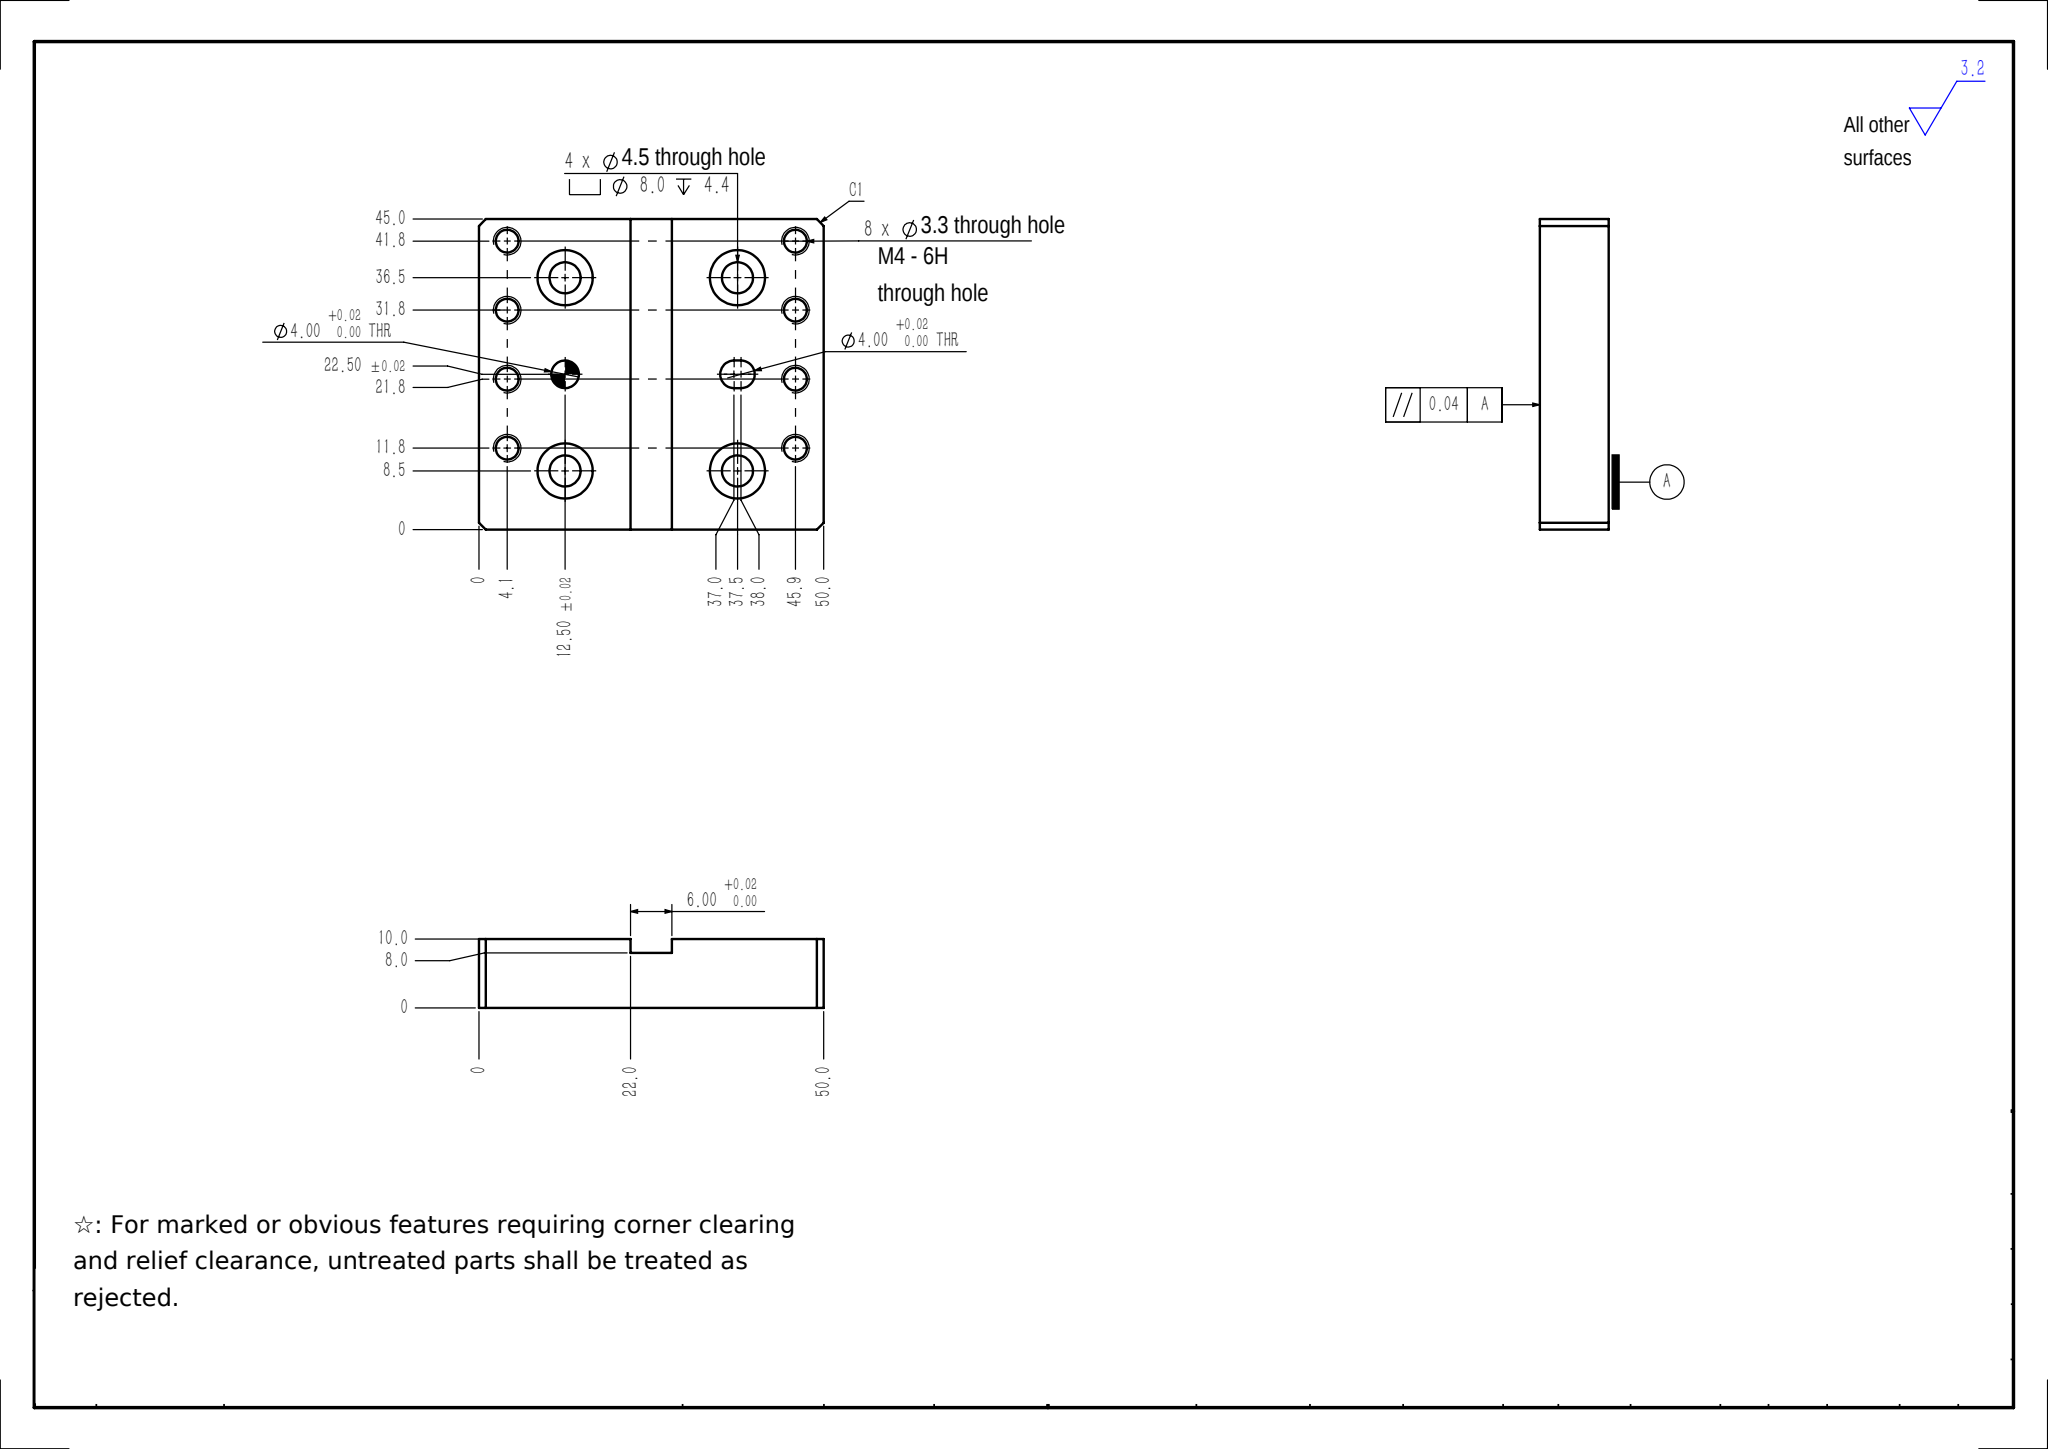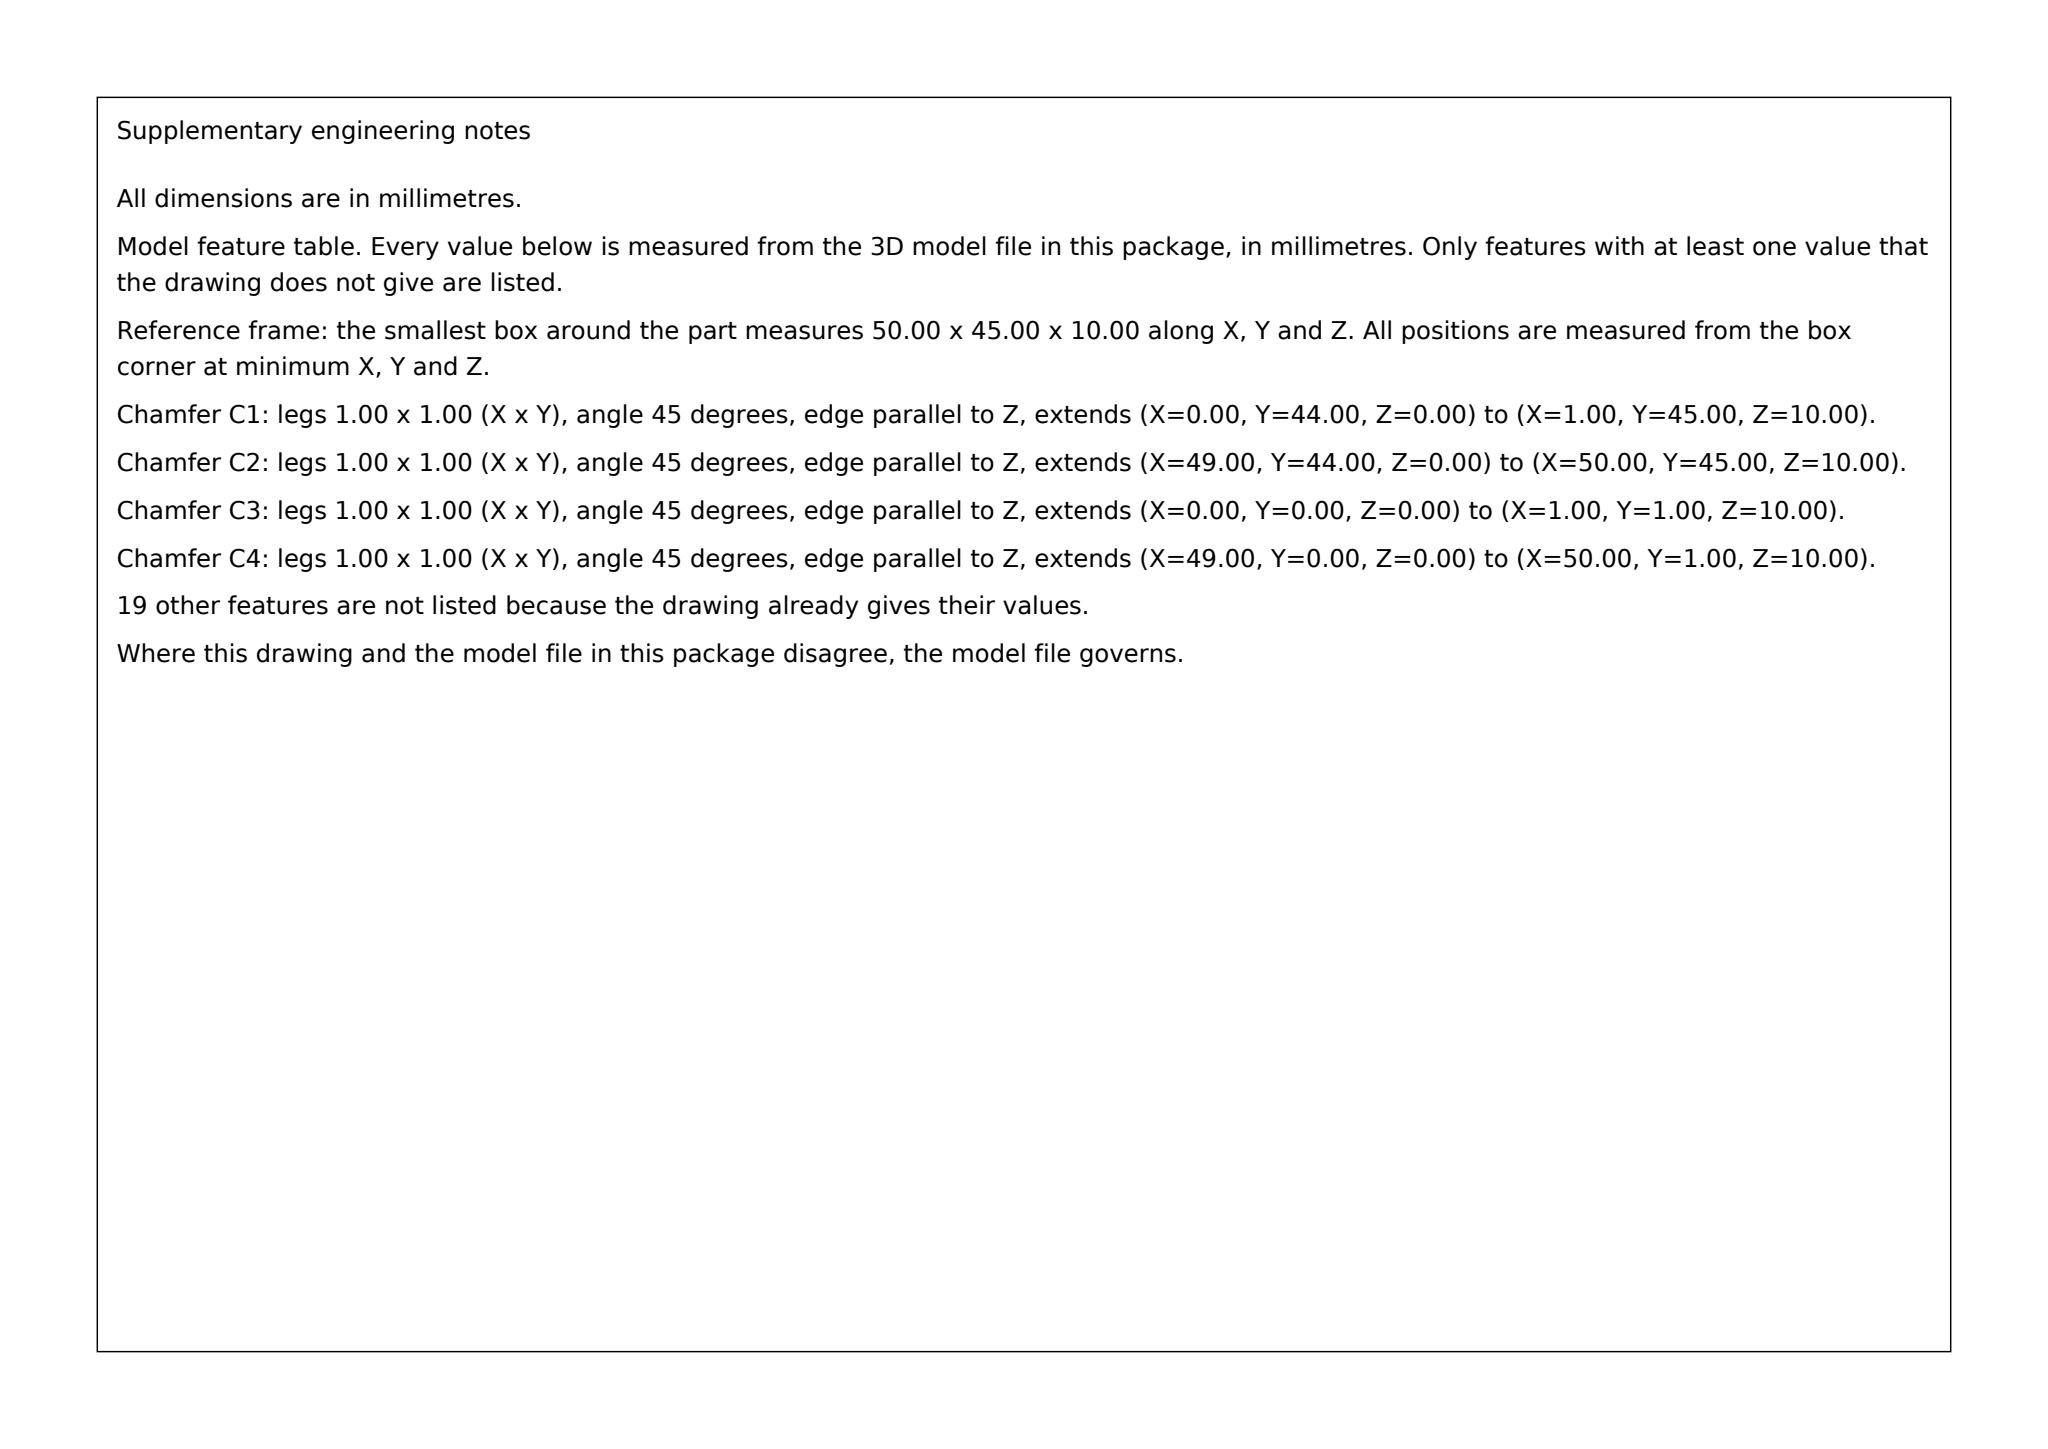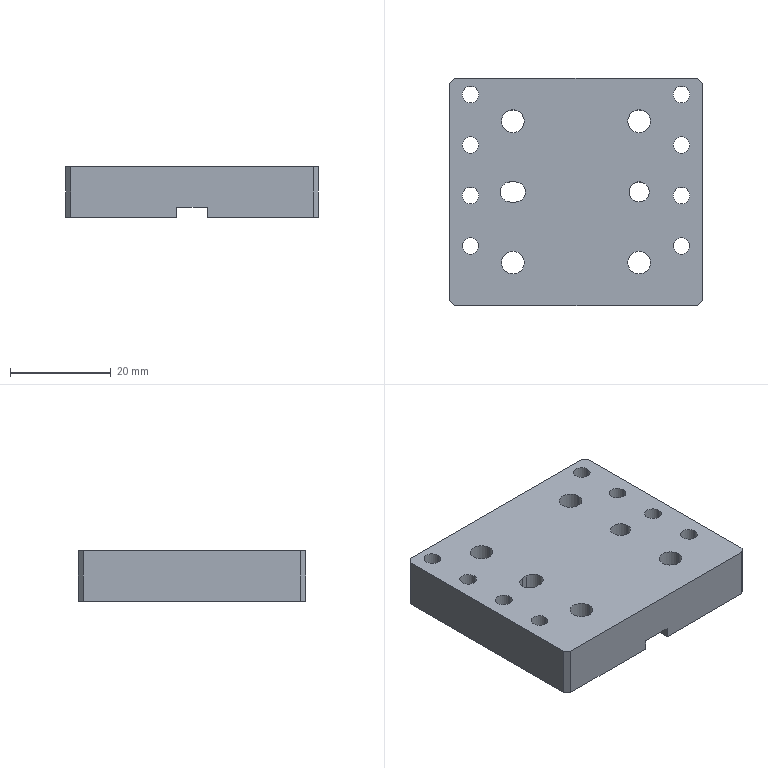Part | SolidWorks | mm | 1 solid | 57 faces | box 50 x 45 x 10 mm | volume 19724 mm3 | cylinder 37 | plane 20 | commonest cylinder face diameters 3.3 x16 8 x8 4.5 x8 4 x5
build123d program:
from build123d import *

# Parameters (mm, degrees)
SKETCH1_W                                       = 50
SKETCH1_H                                       = 45
BOSS_EXTRUDE1_DEPTH                             = 10
M4_HEX_SOCKET_HEAD_CAP_SCREW_CBORE1_D           = 4.5
M4_HEX_SOCKET_HEAD_CAP_SCREW_CBORE1_CBORE_D     = 8
M4_HEX_SOCKET_HEAD_CAP_SCREW_CBORE1_CBORE_DEPTH = 4.4
SKETCH5_R                                       = 2
CUT_EXTRUDE1_DEPTH                              = 36.089
M4_TAPPED_HOLE1_D                               = 3.3
SKETCH8_W                                       = 6
SKETCH8_H                                       = 45
CUT_EXTRUDE2_DEPTH                              = 2
CHAMFER1_SIZE                                   = 1


with BuildPart() as part:
    # Sketch1 → Boss-Extrude1 (new body)
    with BuildSketch(Plane.XY):
        Rectangle(SKETCH1_W, SKETCH1_H)
    extrude(amount=BOSS_EXTRUDE1_DEPTH)

    # M4 Hex Socket Head Cap Screw CBORE1 (through all)
    with Locations(Plane(origin=(0, 0, 0), x_dir=(-1, 0, 0), z_dir=(0, 0, -1))):
        with Locations((12.5, -14), (-12.5, -14), (12.5, 14), (-12.5, 14)):
            CounterBoreHole(M4_HEX_SOCKET_HEAD_CAP_SCREW_CBORE1_D / 2, M4_HEX_SOCKET_HEAD_CAP_SCREW_CBORE1_CBORE_D / 2, M4_HEX_SOCKET_HEAD_CAP_SCREW_CBORE1_CBORE_DEPTH)

    # Sketch5 → Cut-Extrude1 (cut, through all)
    with BuildSketch(Plane(origin=(0, 0, 0), x_dir=(-1, 0, 0), z_dir=(0, 0, -1))):
        with Locations((-12.5, 0)):
            Circle(SKETCH5_R)
        with BuildLine():
            Line((12, 2), (13, 2))
            ThreePointArc((13, 2), (15, 0), (13, -2))
            Line((13, -2), (12, -2))
            ThreePointArc((12, -2), (10, 0), (12, 2))
        make_face()
    extrude(amount=-CUT_EXTRUDE1_DEPTH, mode=Mode.SUBTRACT)

    # M4 Tapped Hole1 (through all)
    with Locations(Plane(origin=(0, 0, 0), x_dir=(-1, 0, 0), z_dir=(0, 0, -1))):
        with Locations((20.9, 19.3), (-20.9, 19.3), (20.9, 9.3), (-20.9, 9.3), (20.9, -0.7), (-20.9, -0.7), (20.9, -10.7), (-20.9, -10.7)):
            Hole(M4_TAPPED_HOLE1_D / 2)

    # Sketch8 → Cut-Extrude2 (cut)
    with BuildSketch(Plane(origin=(0, 0, 0), x_dir=(-1, 0, 0), z_dir=(0, 0, -1))):
        Rectangle(SKETCH8_W, SKETCH8_H)
    extrude(amount=-CUT_EXTRUDE2_DEPTH, mode=Mode.SUBTRACT)

    # Chamfer1
    chamfer1_edges = [part.edges().sort_by_distance(p)[0] for p in [
        (25, -22.5, 5),
        (-25, -22.5, 5),
        (-25, 22.5, 5),
        (25, 22.5, 5),
    ]]
    chamfer(chamfer1_edges, length=CHAMFER1_SIZE)


solid = part.part